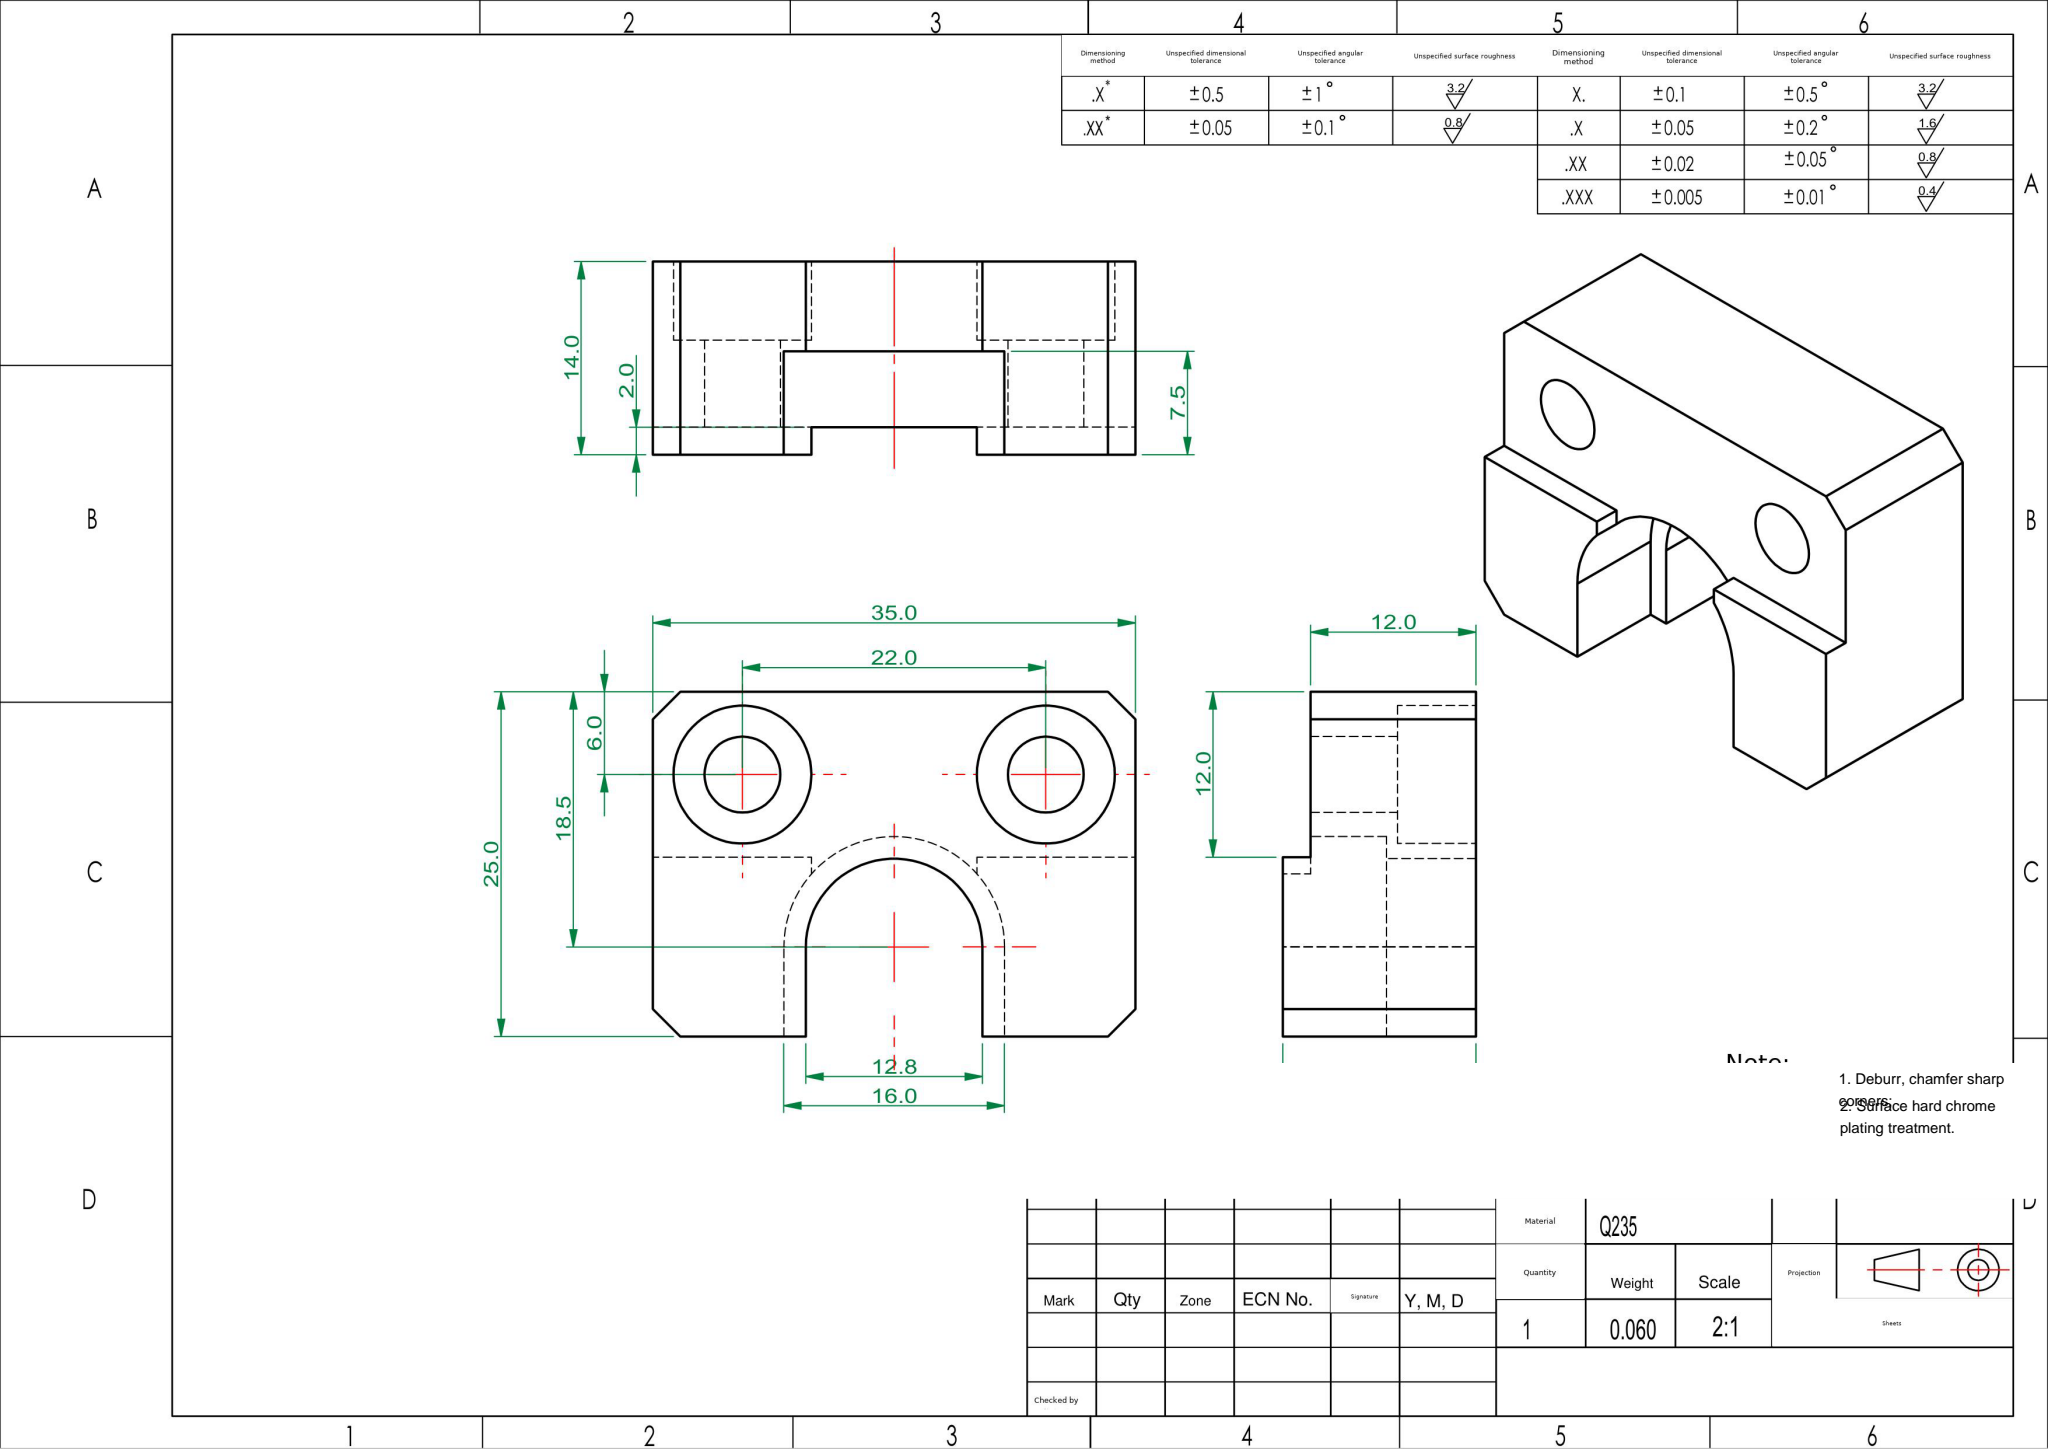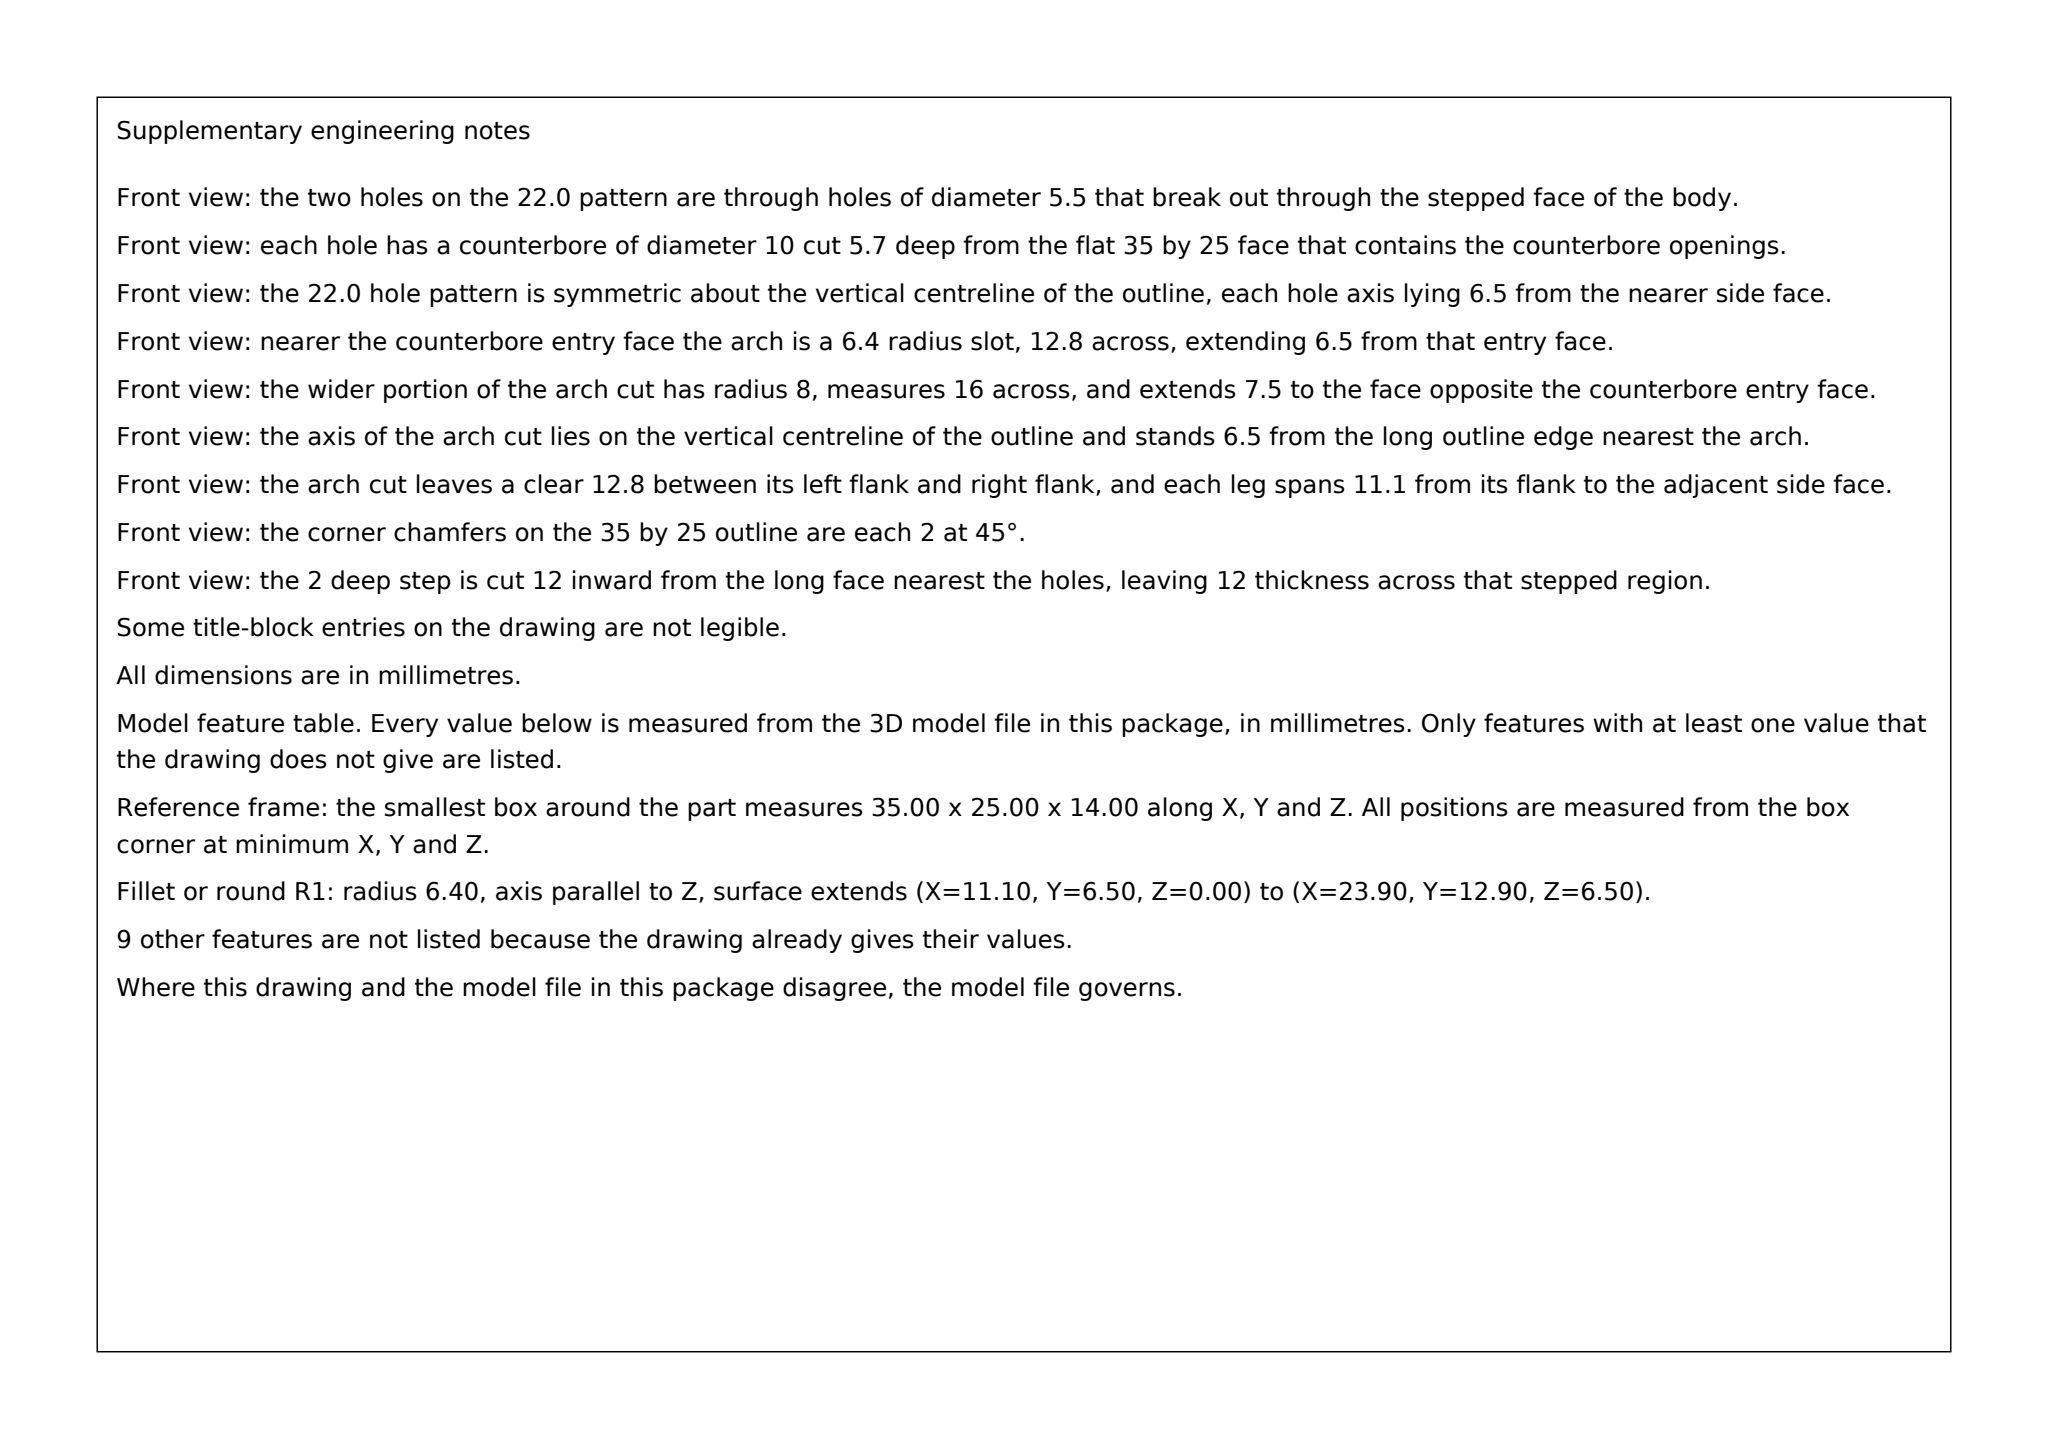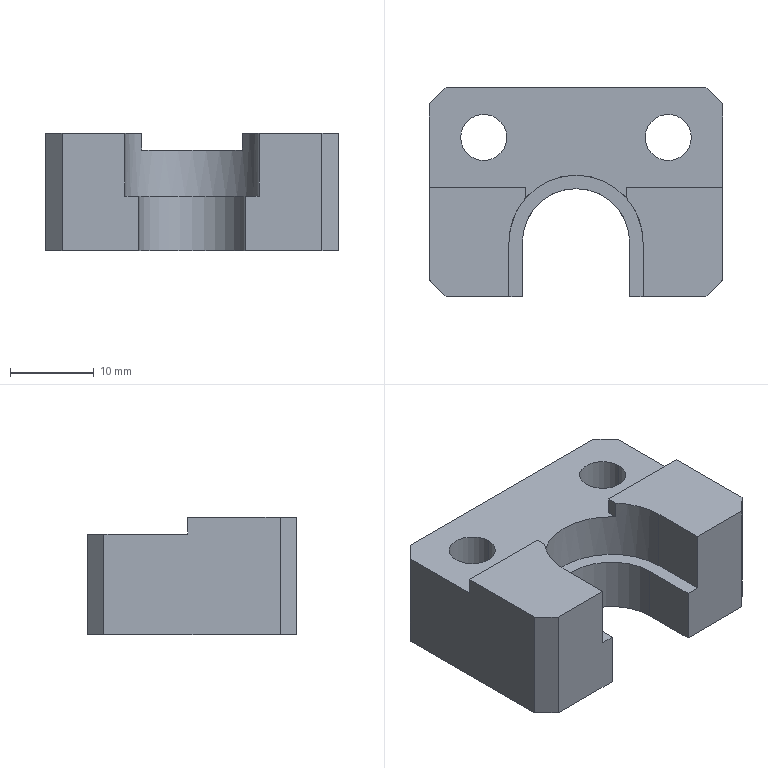Part | SolidWorks | mm | material Q235 | 1 solid | 34 faces | box 35 x 25 x 14 mm | volume 7634 mm3 | plane 24 | cylinder 10 | commonest cylinder face diameters 10 x4 5.5 x4 12.8 x1 16 x1
Drawing notes:
TOP VIEW: 14.0 TO 12.0 THK STEP FACE 13.0 FROM BOTTOM EDGE | from the solid: y-normal planes at 0.0, 13.0, 25.0; thickness z=14.0 for y<13.0, z=12.0 for y>13.0 (two y=13.0 riser faces)
NOTCH 12.0 W x 2.0 DP IN TOP FACE, 13.0 LG FROM BOTTOM EDGE | from the solid: x planes 11.5 & 23.5 (12.0 apart, symm abt x=17.5); z planes 12.0 & 14.0 (2.0 deep); notch runs y=0 to y=13.0 giving two z=14.0 top pads
4: 12.0 = WIDTH OF 2.0 DEEP TOP NOTCH, SYMM ABOUT CL | from the solid: x=23.5 - x=11.5 = 12.0, centered on bbox CL x=17.5 (35.0/2)
2X C'BORE Ø10.0 DP 5.7 FOR Ø5.5 THRU, FROM TOP-VIEW FACE | from the solid: Ø10.0 cyl L=5.7 coaxial with Ø5.5 cyl L=6.3 at (6.5,19.0) and (28.5,19.0); 5.7+6.3=12.0 = local thickness, c'bore opens at z=0 face
build123d program:
from build123d import *

# Parameters (mm, degrees)
SKETCH1_W                                         = 35
SKETCH1_H                                         = 25
BOSS_EXTRUDE1_DEPTH                               = 14
SKETCH2_W                                         = 35
SKETCH2_H                                         = 12
CUT_EXTRUDE1_DEPTH                                = 2
HOLE_SIZE_ACCORDING_TO_HEXAGON_SOCKET_D           = 5.5
HOLE_SIZE_ACCORDING_TO_HEXAGON_SOCKET_CBORE_D     = 10
HOLE_SIZE_ACCORDING_TO_HEXAGON_SOCKET_CBORE_DEPTH = 5.7
CUT_EXTRUDE2_DEPTH                                = 26
CUT_EXTRUDE3_DEPTH                                = 7.5
CHAMFER2_SIZE                                     = 2
SKETCH8_W                                         = 12
SKETCH8_H                                         = 8
CUT_EXTRUDE5_DEPTH                                = 2


with BuildPart() as part:
    # Sketch1 → Boss-Extrude1 (new body)
    with BuildSketch(Plane.XY):
        Rectangle(SKETCH1_W, SKETCH1_H)
    extrude(amount=BOSS_EXTRUDE1_DEPTH)

    # Sketch2 → Cut-Extrude1 (cut)
    with BuildSketch(Plane.XY.offset(14)):
        with Locations((0, 6.5)):
            Rectangle(SKETCH2_W, SKETCH2_H)
    extrude(amount=-CUT_EXTRUDE1_DEPTH, mode=Mode.SUBTRACT)

    # Hole Size _ according to_ Hexagon Socket (through all)
    with Locations(Plane(origin=(11, 6.5, 0), x_dir=(-1, 0, 0), z_dir=(0, 0, -1))):
        with Locations((0, 0), (22, 0)):
            CounterBoreHole(HOLE_SIZE_ACCORDING_TO_HEXAGON_SOCKET_D / 2, HOLE_SIZE_ACCORDING_TO_HEXAGON_SOCKET_CBORE_D / 2, HOLE_SIZE_ACCORDING_TO_HEXAGON_SOCKET_CBORE_DEPTH)

    # Sketch5 → Cut-Extrude2 (cut)
    with BuildSketch(Plane(origin=(0, 0, 0), x_dir=(-1, 0, 0), z_dir=(0, 0, -1))):
        with BuildLine():
            Line((-6.4, -12.5), (-6.4, -6))
            ThreePointArc((-6.4, -6), (0, 0.4), (6.4, -6))
            Line((6.4, -6), (6.4, -12.5))
            ThreePointArc((6.4, -12.5), (0, -18.9), (-6.4, -12.5))
        make_face()
    extrude(amount=-CUT_EXTRUDE2_DEPTH, mode=Mode.SUBTRACT)

    # Sketch6 → Cut-Extrude3 (cut)
    with BuildSketch(Plane.XY.offset(14)):
        with BuildLine():
            Line((8, -6), (8, -12.5))
            ThreePointArc((8, -12.5), (0, -20.5), (-8, -12.5))
            Line((-8, -12.5), (-8, -6))
            ThreePointArc((-8, -6), (0, 2), (8, -6))
        make_face()
    extrude(amount=-CUT_EXTRUDE3_DEPTH, mode=Mode.SUBTRACT)

    # Chamfer2
    chamfer2_edges = [part.edges().sort_by_distance(p)[0] for p in [
        (-17.5, 12.5, 6),
        (17.5, 12.5, 6),
        (17.5, -12.5, 7),
        (-17.5, -12.5, 7),
    ]]
    chamfer(chamfer2_edges, length=CHAMFER2_SIZE)

    # Sketch8 → Cut-Extrude5 (cut)
    with BuildSketch(Plane.XY.offset(14)):
        Rectangle(SKETCH8_W, SKETCH8_H)
    extrude(amount=-CUT_EXTRUDE5_DEPTH, mode=Mode.SUBTRACT)


solid = part.part